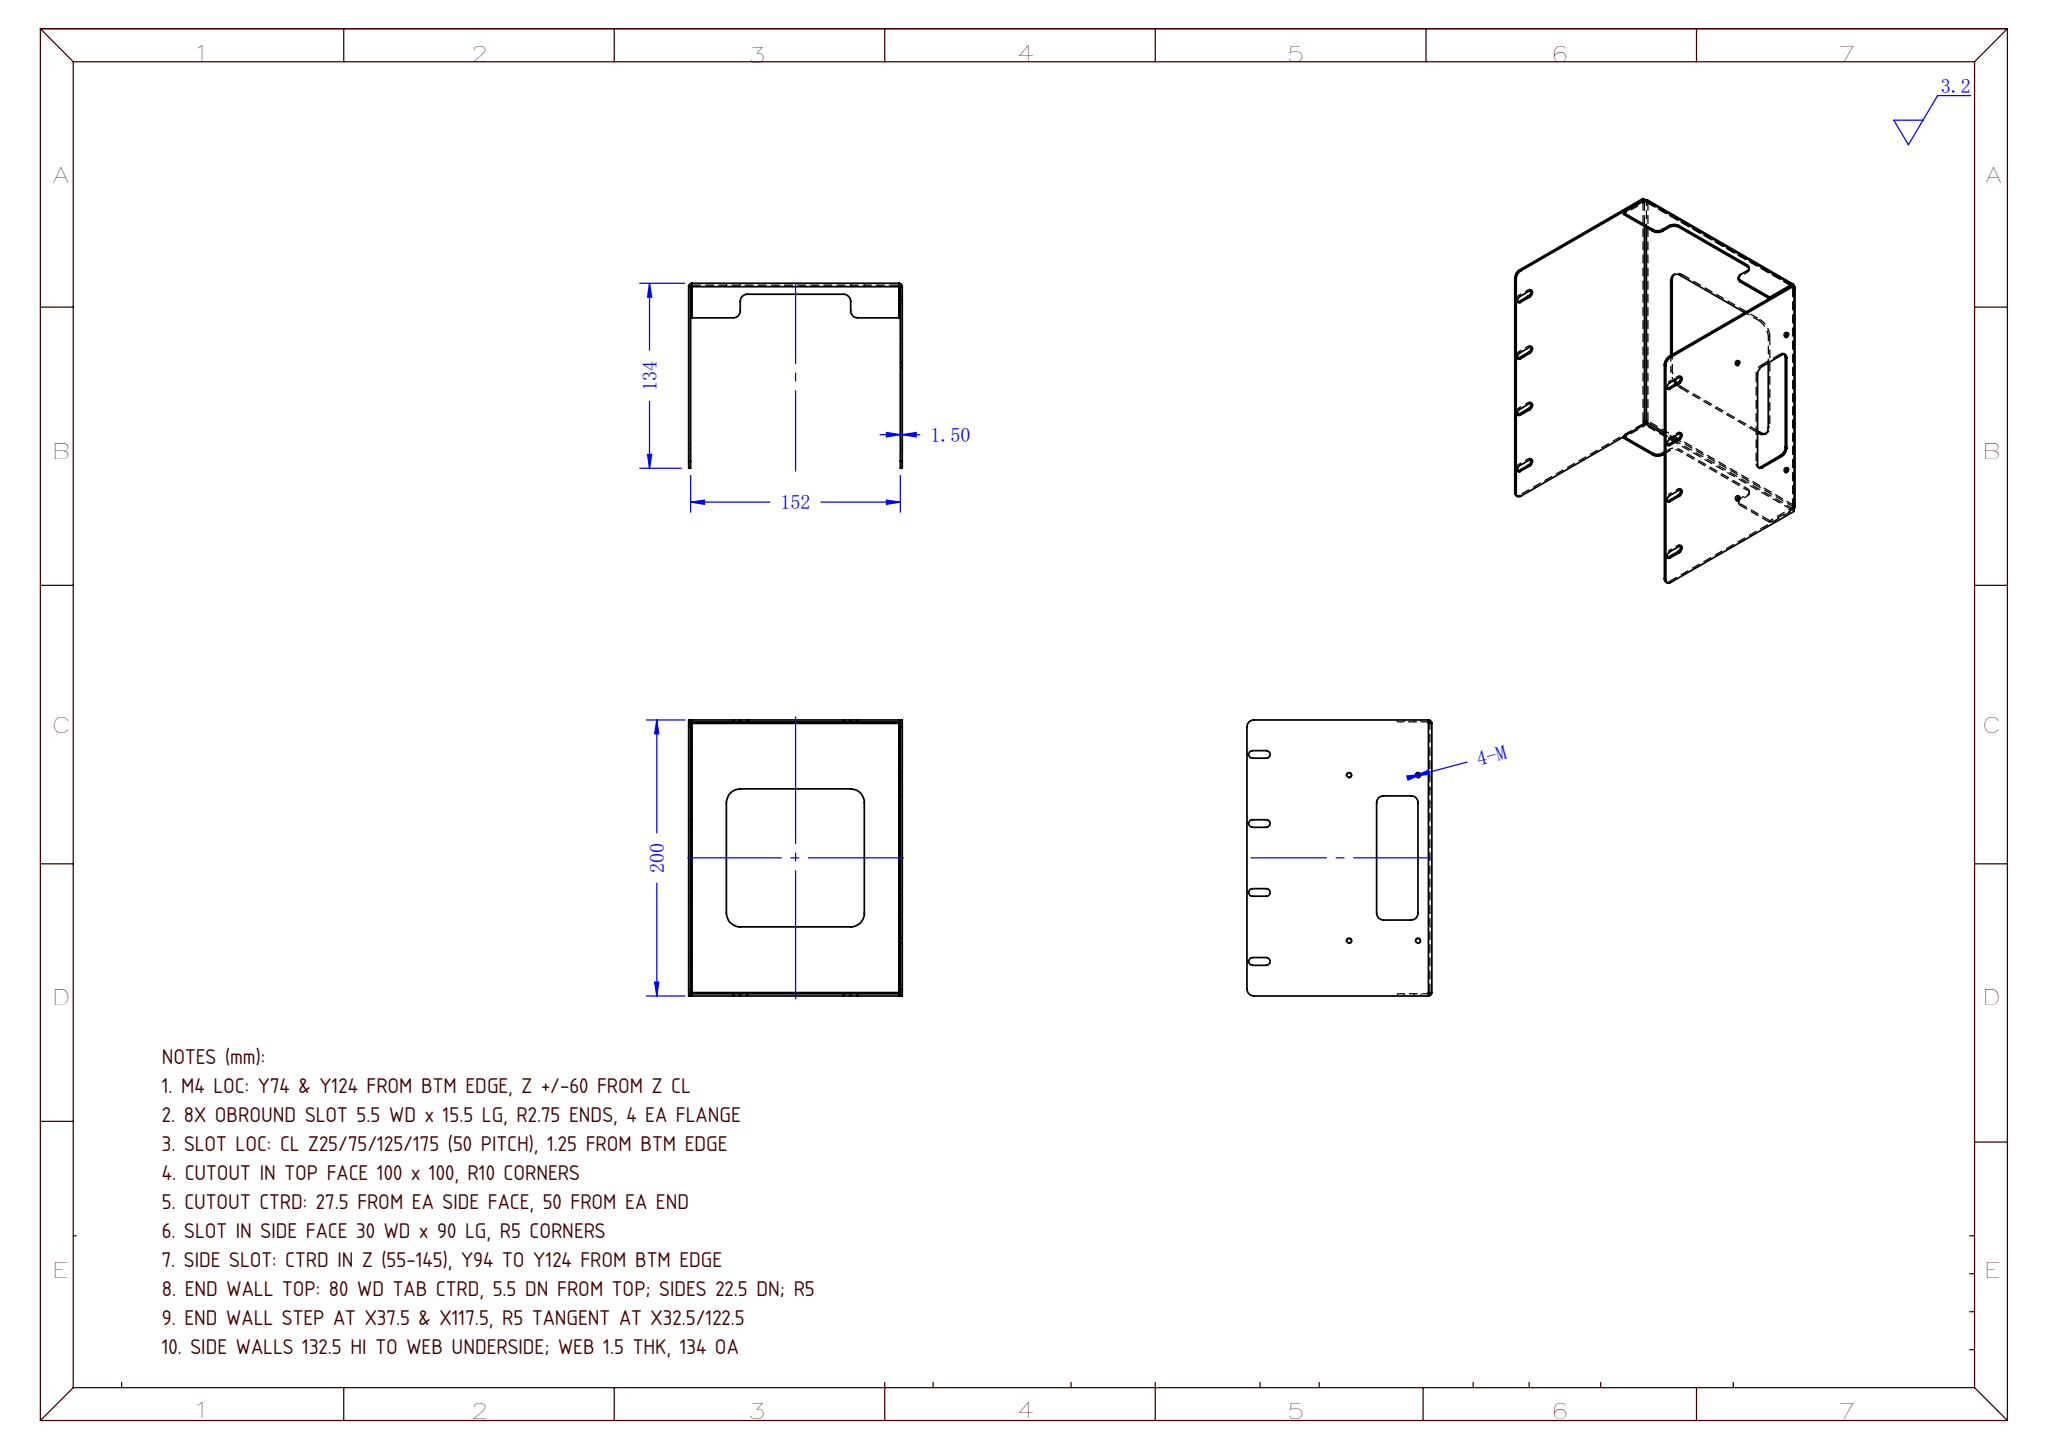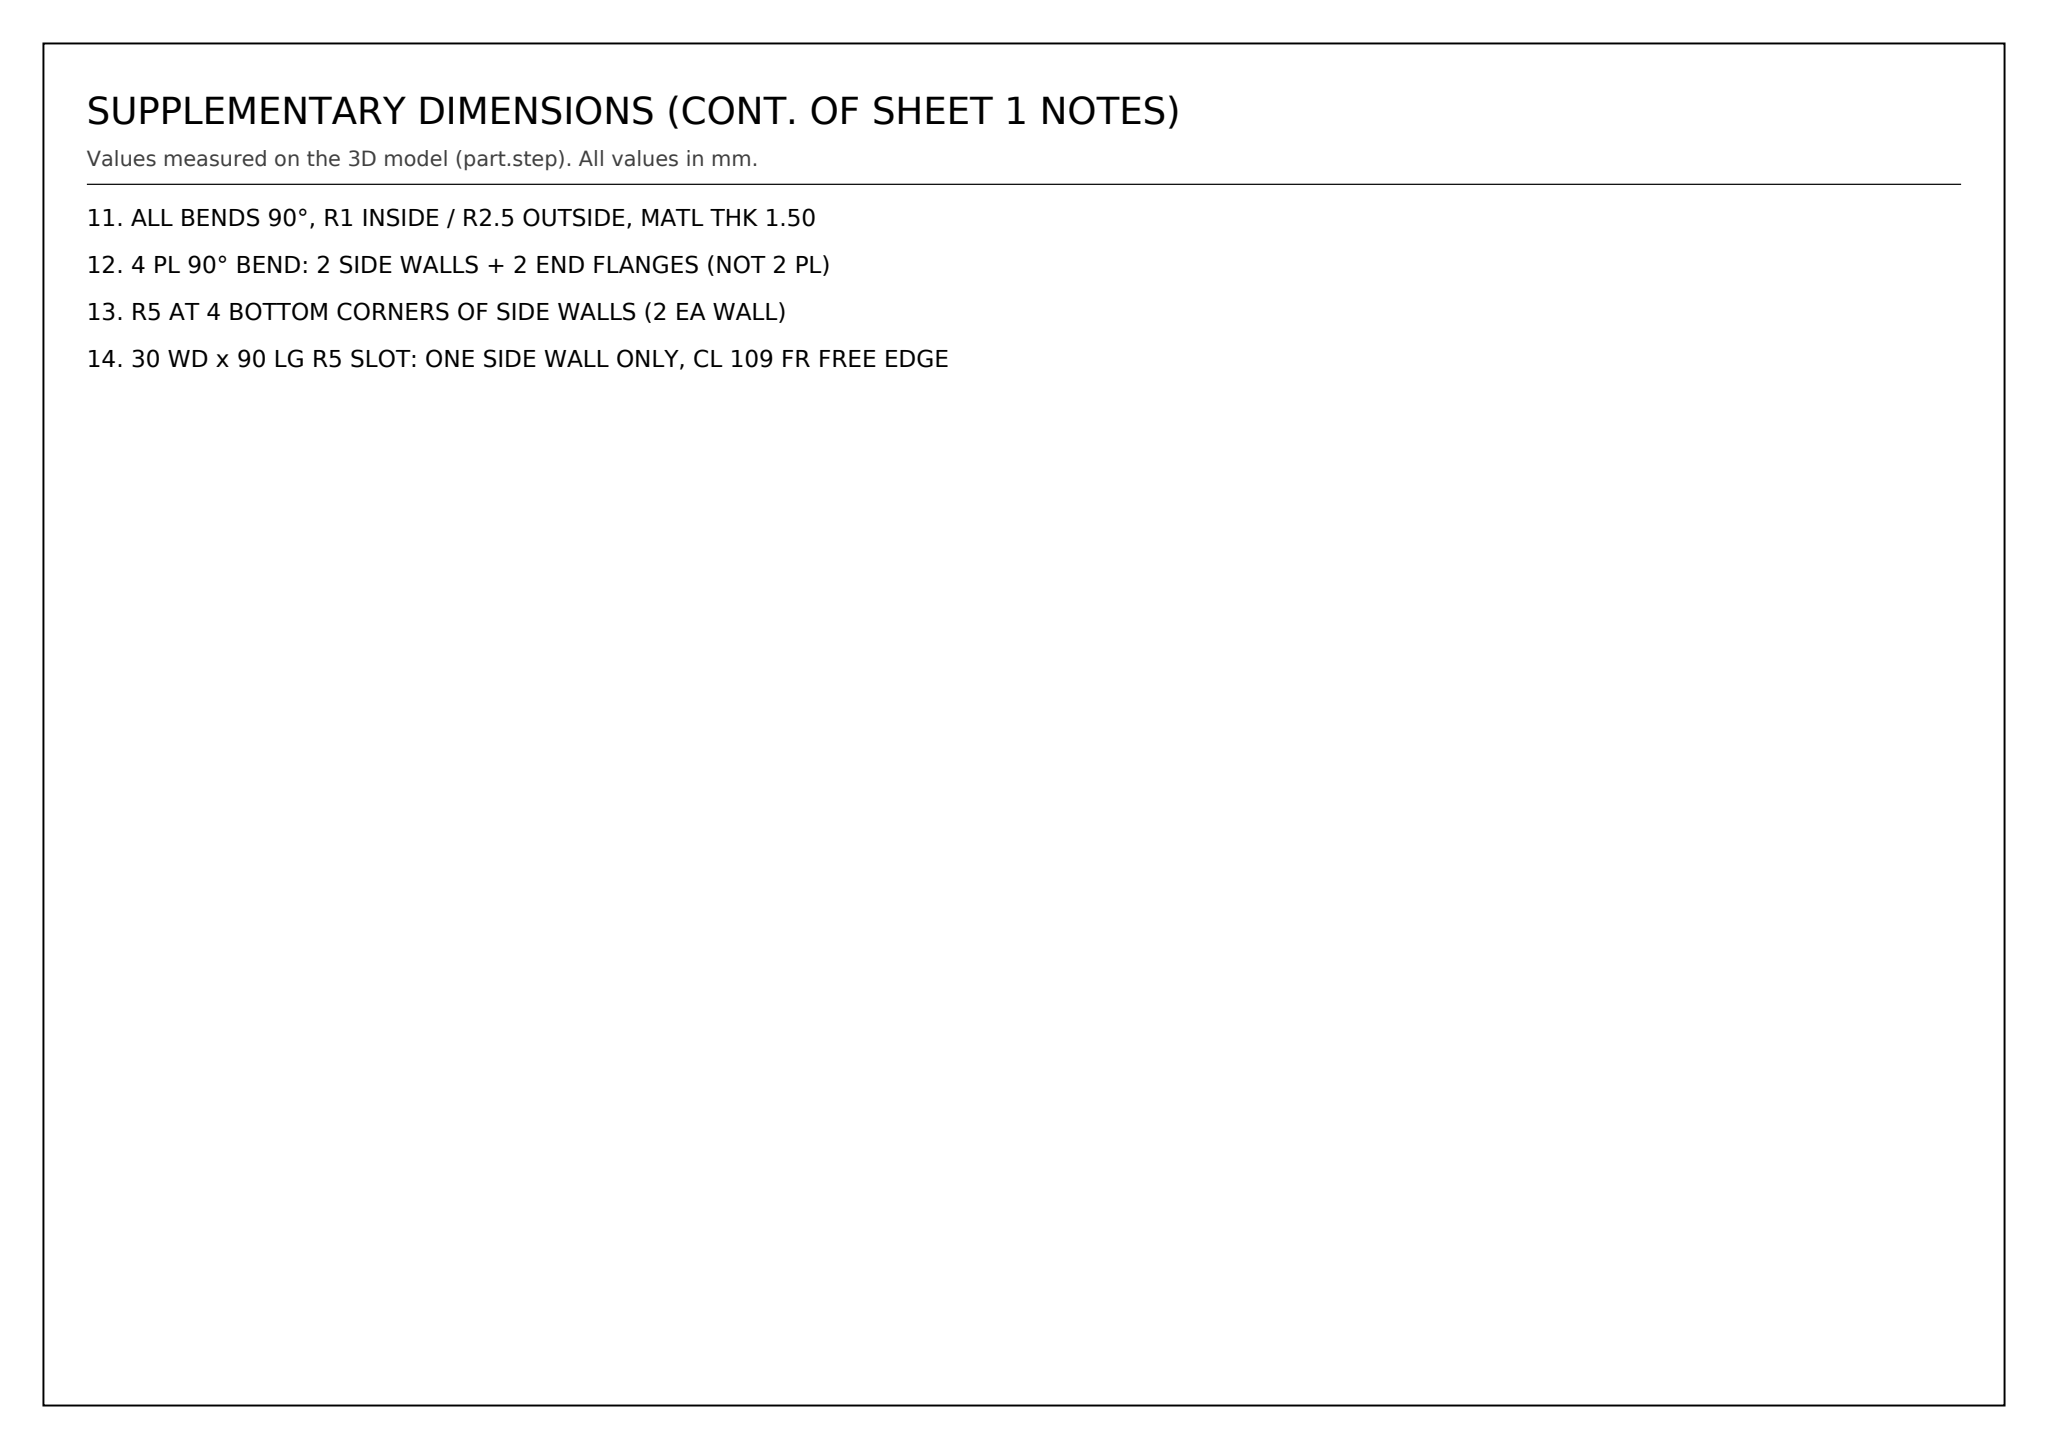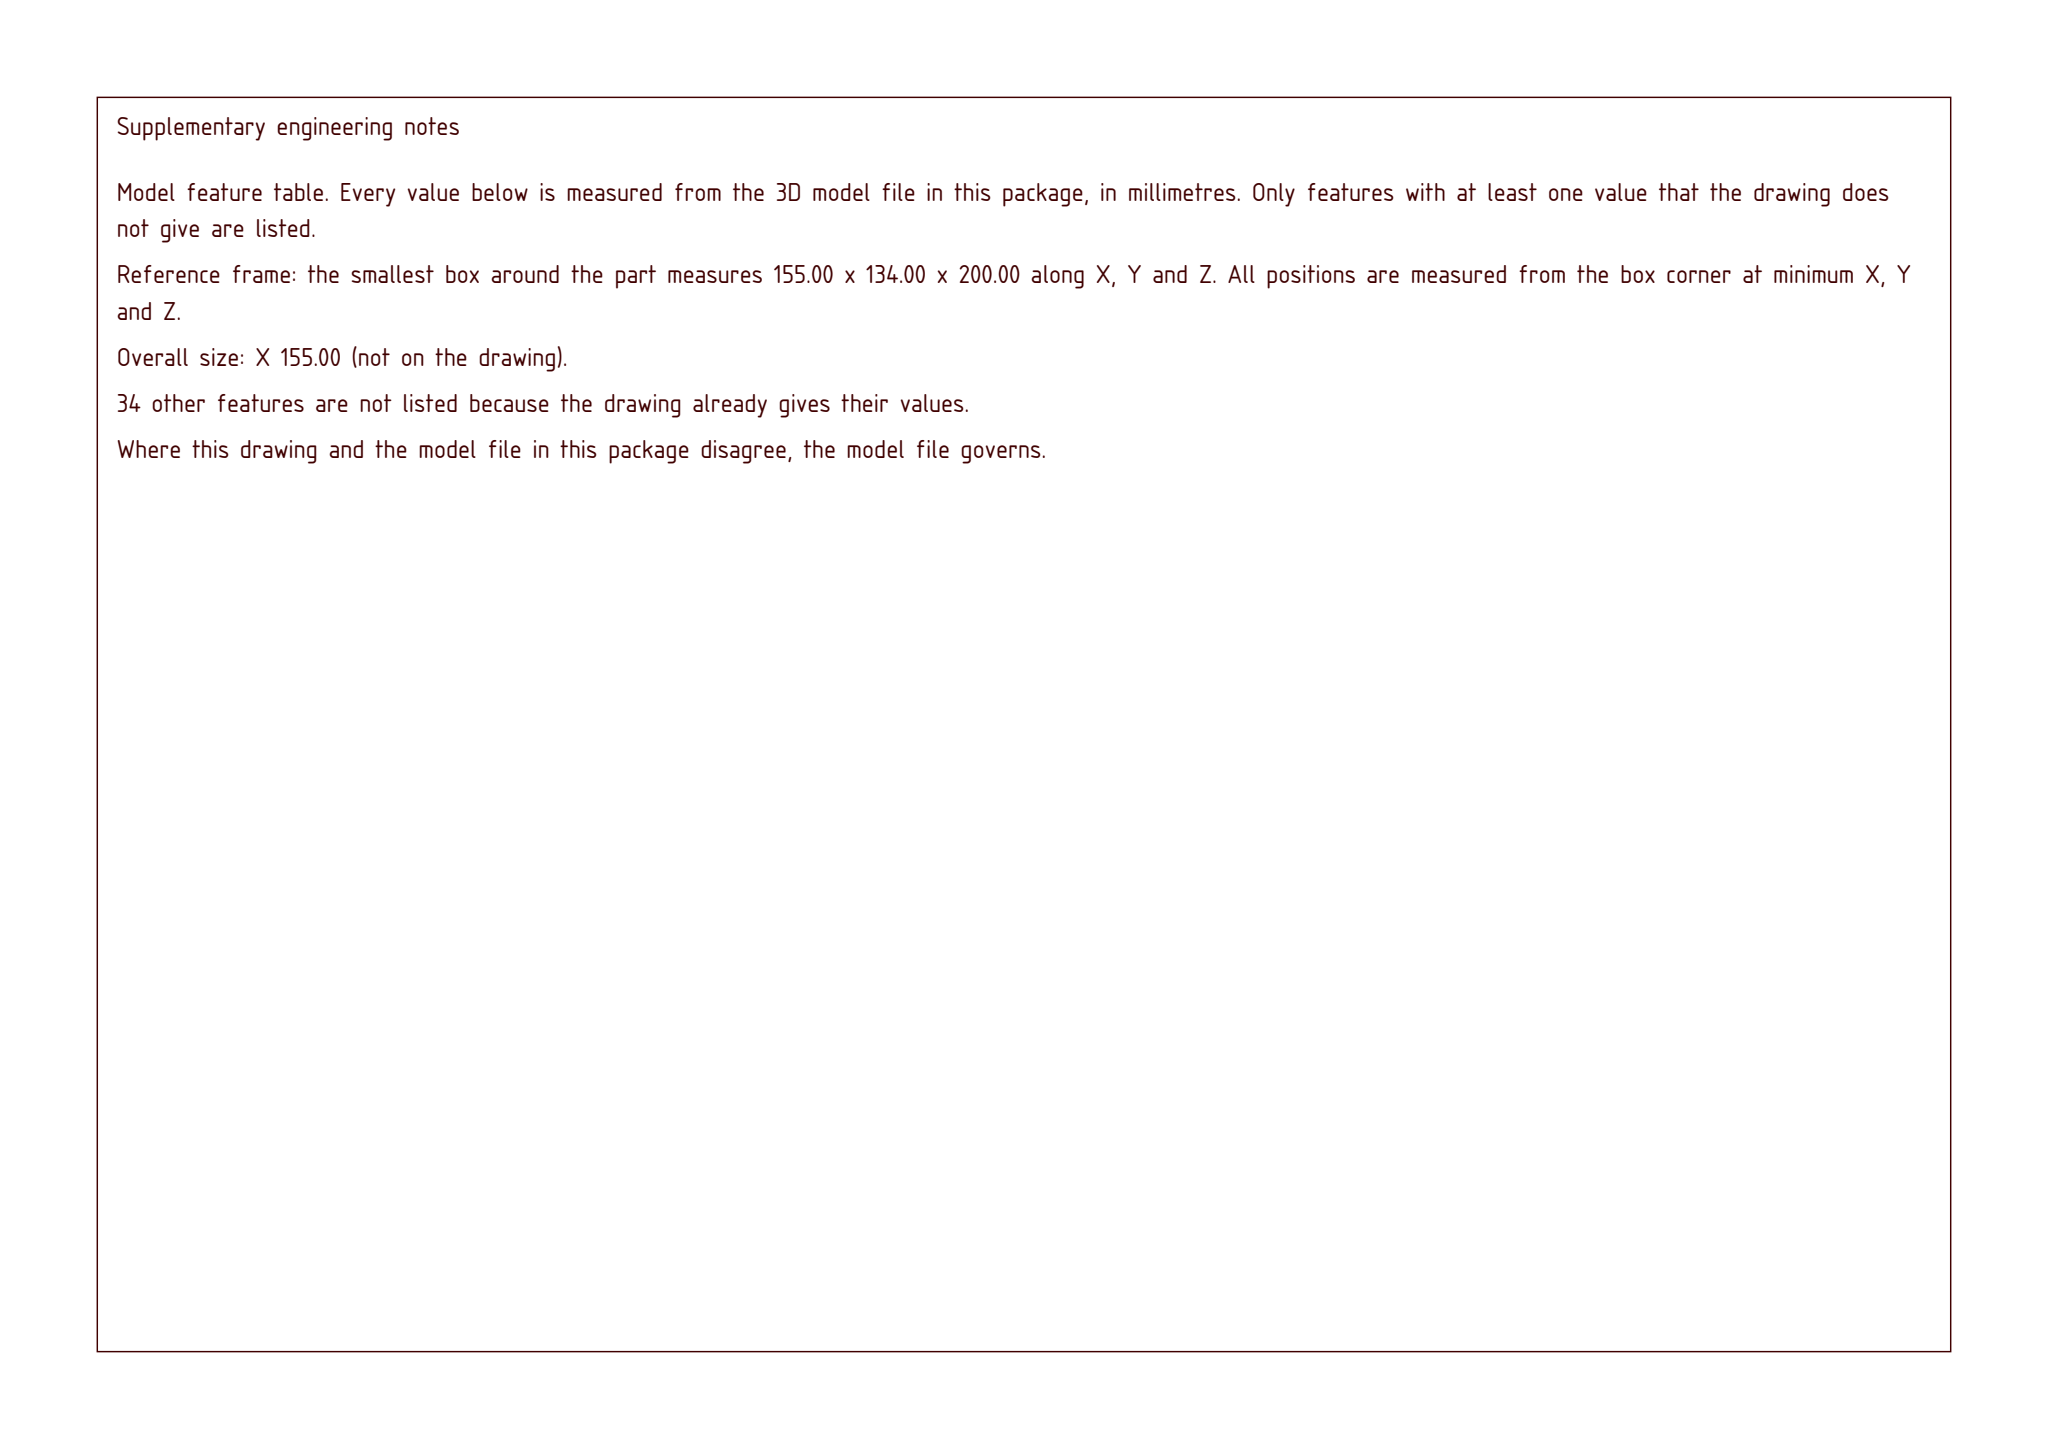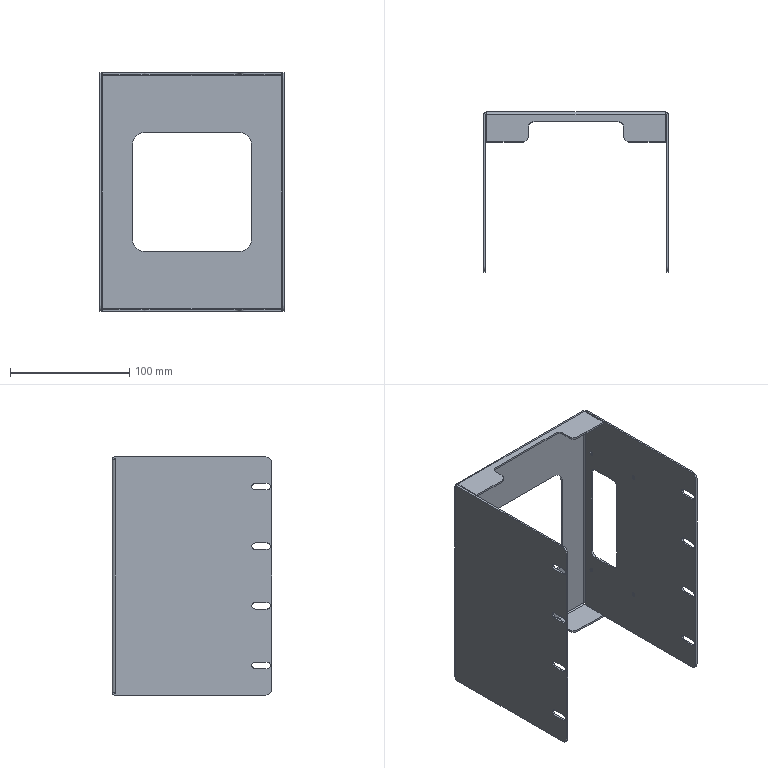Part | SolidWorks | mm | 1 solid | 126 faces | box 155 x 134 x 200 mm | volume 111747 mm3 | plane 66 | cylinder 60 | commonest cylinder face diameters 5.5 x24 10 x16 3.3 x8 5 x4 2 x4 20 x4
Drawing notes:
M4 LOC: Y74 & Y124 FROM BTM EDGE, Z +/-60 FROM Z CL | from the solid: Ø3.3 at y=74/124 (50 apart), z=40/160 about z CL=100 of 200
8X OBROUND SLOT 5.5 WD x 15.5 LG, R2.75 ENDS, 4 EA FLANGE | from the solid: Ø5.5 x 1.5 end radii at y=4 & y=14 (10 apart) => 15.5 oa, 4 z-positions, 2 walls
SLOT LOC: CL Z25/75/125/175 (50 PITCH), 1.25 FROM BTM EDGE | from the solid: Ø5.5 slots at z=25,75,125,175; y=4 end ctr - R2.75 = 1.25 from y=0
CUTOUT IN TOP FACE 100 x 100, R10 CORNERS | from the solid: Ø20 (R10) y-axis cyls at x=37.5/117.5, z=60/140 => 27.5-127.5 x 50-150
CUTOUT CTRD: 27.5 FROM EA SIDE FACE, 50 FROM EA END | from the solid: cutout x 27.5-127.5 of 155, z 50-150 of 200 (planes x27.5/127.5, z50/150)
SLOT IN SIDE FACE 30 WD x 90 LG, R5 CORNERS | from the solid: Ø10 x-axis cyls at y=99/119, z=60/140 => y 94-124, z 55-145
SIDE SLOT: CTRD IN Z (55-145), Y94 TO Y124 FROM BTM EDGE | from the solid: planes y94, y124, z55, z145; z ctr 100 = 200/2
END WALL TOP: 80 WD TAB CTRD, 5.5 DN FROM TOP; SIDES 22.5 DN; R5 | from the solid: End flange plate (z 0-1.5 / 198.5-200) spans y 109 to 131.5; mid recess face y=126 over x 42.5-112.5 (between step faces x37.5 & x117.5 = 80 wd, ctrd on x77.5) -> 131.5-126 = 5.5 dn; outer bottom edge y=109 over x2.5-32.5 & x122.5-152.5 -> 131.5-109 = 22.5 dn; R5 (dia 10) arcs at corners
END WALL STEP AT X37.5 & X117.5, R5 TANGENT AT X32.5/122.5 | from the solid: Vertical step faces x=37.5 and x=117.5 (y 114-121, z 0-1.5); convex R5 arcs (dia 10, axis z) centered at x=32.5 and x=122.5, y=114, tangent to y=109 edge at x32.5/122.5 and to the x37.5/117.5 faces
SIDE WALLS 132.5 HI TO WEB UNDERSIDE; WEB 1.5 THK, 134 OA | from the solid: y planes 0, 132.5, 134; wall thk 1.5 (x 0-1.5, 153.5-155)
ALL BENDS 90°, R1 INSIDE / R2.5 OUTSIDE, MATL THK 1.50 | from the solid: Concave arcs D2.0 (R1) at x=2.5/152.5 & z=2.5/197.5 and convex arcs D5.0 (R2.5) at same bend lines; walls 1.5 thk
4 PL 90° BEND: 2 SIDE WALLS + 2 END FLANGES (NOT 2 PL) | from the solid: Web plane y=132.5/134 (x2.5-152.5, z2.5-197.5) joins walls x=0-1.5 & x=153.5-155 and end flanges z=0-1.5 & z=198.5-200, each via R1/R2.5 bend arcs
R5 AT 4 BOTTOM CORNERS OF SIDE WALLS (2 EA WALL) | from the solid: Convex arcs D10 (R5), axis x, at (y=5,z=5) & (y=5,z=195), each on x=0-1.5 and x=153.5-155
30 WD x 90 LG R5 SLOT: ONE SIDE WALL ONLY, CL 109 FR FREE EDGE | from the solid: Slot faces y=94 & y=124 (30 wd), ends z=55/145 (90 lg), R5 corner arcs D10 at y=99/119, z=60/140, all on wall x=153.5-155 only; CL y=109 from y=0 edge